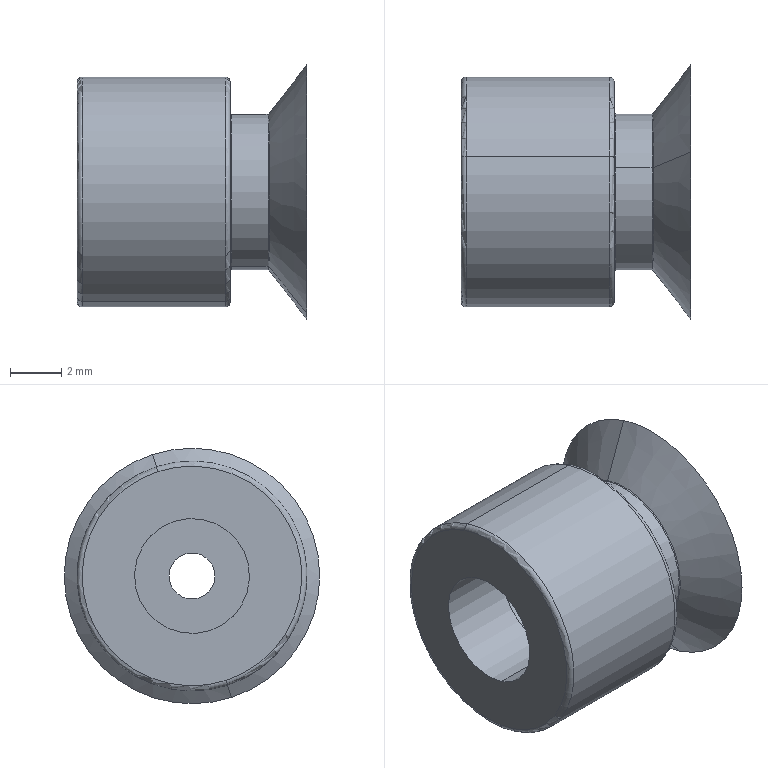Component | SolidWorks | SmallSuctionNozzle-1 | 1 solid | 28 faces | box 9 x 10 x 10 mm | volume 304 mm3 | cylinder 10 | torus 8 | plane 6 | cone 4 | commonest cylinder face diameters 7 x2 1.8 x2 4.5 x2 6.1 x2 9 x2
build123d program:
from build123d import *

# Parameters (mm, degrees)
SKETCH1_R           = 4.5
BOSS_EXTRUDE1_DEPTH = 3
SKETCH2_R           = 3.05
BOSS_EXTRUDE2_DEPTH = 1.5
SKETCH4_R           = 2.25
CUT_EXTRUDE1_DEPTH  = 5.5
SKETCH6_R           = 0.9
CUT_EXTRUDE3_DEPTH  = 11.308
SKETCH7_R           = 3.5
CUT_EXTRUDE6_DEPTH  = 2.5
FILLET1_R           = 0.2
FILLET2_R           = 0.05


with BuildPart() as part:
    # Sketch1 → Boss-Extrude1 (new, symmetric)
    with BuildSketch(Plane.XY):
        Circle(SKETCH1_R)
    extrude(amount=BOSS_EXTRUDE1_DEPTH, both=True)

    # Sketch2 → Boss-Extrude2 (add)
    with BuildSketch(Plane.XY.offset(3)):
        Circle(SKETCH2_R)
    extrude(amount=BOSS_EXTRUDE2_DEPTH)

    # Sketch3 → Revolve1 (revolve)
    with BuildSketch(Plane(origin=(0, 0, 0), x_dir=(1, 0, 0), z_dir=(0, 1, 0)), mode=Mode.PRIVATE) as revolve1_sk:
        Polygon((-4.18, -6), (-2.23, -4.5), (-3.05, -4.5), (-5, -6), align=None)
    revolve(revolve1_sk.sketch.rotate(Axis((0, 0, -3), (0, 0, 1)), 180), axis=Axis((0, 0, -3), (0, 0, 1)))

    # Sketch4 → Cut-Extrude1 (cut)
    with BuildSketch(Plane(origin=(0, 0, -3), x_dir=(-1, 0, 0), z_dir=(0, 0, -1))):
        Circle(SKETCH4_R)
    extrude(amount=-CUT_EXTRUDE1_DEPTH, mode=Mode.SUBTRACT)

    # Sketch6 → Cut-Extrude3 (cut, through all)
    with BuildSketch(Plane.XY.offset(4.5)):
        Circle(SKETCH6_R)
    extrude(amount=-CUT_EXTRUDE3_DEPTH, mode=Mode.SUBTRACT)

    # Sketch7 → Cut-Extrude6 (cut)
    with BuildSketch(Plane(origin=(0, 0, 2.5), x_dir=(-1, 0, 0), z_dir=(0, 0, -1))):
        Circle(SKETCH7_R)
    extrude(amount=CUT_EXTRUDE6_DEPTH, mode=Mode.SUBTRACT)

    # Fillet1
    fillet1_edges = [part.edges().sort_by_distance(p)[0] for p in [
        (-4.5, 0, -3),
        (-4.5, 0, 3),
    ]]
    fillet(fillet1_edges, radius=FILLET1_R)

    # Fillet2
    fillet2_edges = [part.edges().sort_by_distance(p)[0] for p in [
        (-3.05, 0, 3),
        (-3.05, 0, 4.5),
    ]]
    fillet(fillet2_edges, radius=FILLET2_R)


solid = part.part

# Placed as in the assembly
solid = solid.moved(Location((-558.696, -21.651, 373.468), (0, 90, 0)))
STEP:
#1=COLOUR_RGB('',0.7922,0.8196,0.9333);
#2=FILL_AREA_STYLE_COLOUR('',#1);
#3=FILL_AREA_STYLE('',(#2));
#4=SURFACE_STYLE_FILL_AREA(#3);
#5=SURFACE_SIDE_STYLE('',(#4));
#6=SURFACE_STYLE_USAGE(.BOTH.,#5);
#7=PRESENTATION_STYLE_ASSIGNMENT((#6));
#8=CARTESIAN_POINT('',(-21.818,-0.8149,14.818));
#9=VERTEX_POINT('',#8);
#10=CARTESIAN_POINT('',(-21.818,-0.8899,14.589));
#11=VERTEX_POINT('',#10);
#12=CARTESIAN_POINT('',(-21.818,-0.8524,14.703));
#13=DIRECTION('',(1.,-0.,0.));
#14=DIRECTION('',(0.,0.3102,0.9507));
#15=AXIS2_PLACEMENT_3D('',#12,#13,#14);
#16=CIRCLE('',#15,0.1208);
#17=EDGE_CURVE('',#9,#11,#16,.T.);
#18=ORIENTED_EDGE('',*,*,#17,.F.);
#19=CARTESIAN_POINT('',(-21.82,-0.8152,14.818));
#20=VERTEX_POINT('',#19);
#21=CARTESIAN_POINT('',(-21.82,-0.8146,14.819));
#22=DIRECTION('',(0.,0.9507,-0.3102));
#23=DIRECTION('',(0.,0.3102,0.9507));
#24=AXIS2_PLACEMENT_3D('',#21,#22,#23);
#25=CIRCLE('',#24,0.001969);
#26=EDGE_CURVE('',#9,#20,#25,.T.);
#27=ORIENTED_EDGE('',*,*,#26,.T.);
#28=CARTESIAN_POINT('',(-21.82,-0.8897,14.589));
#29=VERTEX_POINT('',#28);
#30=CARTESIAN_POINT('',(-21.82,-0.8524,14.703));
#31=DIRECTION('',(-1.,0.,-0.));
#32=DIRECTION('',(0.,-0.3102,-0.9507));
#33=AXIS2_PLACEMENT_3D('',#30,#31,#32);
#34=CIRCLE('',#33,0.1201);
#35=EDGE_CURVE('',#29,#20,#34,.T.);
#36=ORIENTED_EDGE('',*,*,#35,.F.);
#37=CARTESIAN_POINT('',(-21.82,-0.8903,14.587));
#38=DIRECTION('',(-0.,-0.9507,0.3102));
#39=DIRECTION('',(0.,-0.3102,-0.9507));
#40=AXIS2_PLACEMENT_3D('',#37,#38,#39);
#41=CIRCLE('',#40,0.001969);
#42=EDGE_CURVE('',#11,#29,#41,.T.);
#43=ORIENTED_EDGE('',*,*,#42,.F.);
#44=EDGE_LOOP('',(#18,#27,#36,#43));
#45=FACE_OUTER_BOUND('',#44,.T.);
#46=CARTESIAN_POINT('',(-21.82,-0.8524,14.703));
#47=DIRECTION('',(1.,-0.,0.));
#48=DIRECTION('',(0.,-0.3102,-0.9507));
#49=AXIS2_PLACEMENT_3D('',#46,#47,#48);
#50=TOROIDAL_SURFACE('',#49,0.122,0.001969);
#51=ADVANCED_FACE('',(#45),#50,.F.);
#52=CARTESIAN_POINT('',(-21.876,-0.8152,14.818));
#53=VERTEX_POINT('',#52);
#54=CARTESIAN_POINT('',(-21.876,-0.8897,14.589));
#55=VERTEX_POINT('',#54);
#56=CARTESIAN_POINT('',(-21.876,-0.8524,14.703));
#57=DIRECTION('',(1.,-0.,0.));
#58=DIRECTION('',(0.,-0.3102,-0.9507));
#59=AXIS2_PLACEMENT_3D('',#56,#57,#58);
#60=CIRCLE('',#59,0.1201);
#61=EDGE_CURVE('',#53,#55,#60,.T.);
#62=ORIENTED_EDGE('',*,*,#61,.F.);
#63=CARTESIAN_POINT('',(-21.878,-0.8146,14.819));
#64=VERTEX_POINT('',#63);
#65=CARTESIAN_POINT('',(-21.876,-0.8146,14.819));
#66=DIRECTION('',(0.,0.9507,-0.3102));
#67=DIRECTION('',(0.,0.3102,0.9507));
#68=AXIS2_PLACEMENT_3D('',#65,#66,#67);
#69=CIRCLE('',#68,0.001969);
#70=EDGE_CURVE('',#53,#64,#69,.T.);
#71=ORIENTED_EDGE('',*,*,#70,.T.);
#72=CARTESIAN_POINT('',(-21.878,-0.8903,14.587));
#73=VERTEX_POINT('',#72);
#74=CARTESIAN_POINT('',(-21.878,-0.8524,14.703));
#75=DIRECTION('',(-1.,0.,-0.));
#76=DIRECTION('',(0.,-0.3102,-0.9507));
#77=AXIS2_PLACEMENT_3D('',#74,#75,#76);
#78=CIRCLE('',#77,0.122);
#79=EDGE_CURVE('',#73,#64,#78,.T.);
#80=ORIENTED_EDGE('',*,*,#79,.F.);
#81=CARTESIAN_POINT('',(-21.876,-0.8903,14.587));
#82=DIRECTION('',(-0.,-0.9507,0.3102));
#83=DIRECTION('',(0.,-0.3102,-0.9507));
#84=AXIS2_PLACEMENT_3D('',#81,#82,#83);
#85=CIRCLE('',#84,0.001969);
#86=EDGE_CURVE('',#55,#73,#85,.T.);
#87=ORIENTED_EDGE('',*,*,#86,.F.);
#88=EDGE_LOOP('',(#62,#71,#80,#87));
#89=FACE_OUTER_BOUND('',#88,.T.);
#90=CARTESIAN_POINT('',(-21.876,-0.8524,14.703));
#91=DIRECTION('',(1.,-0.,0.));
#92=DIRECTION('',(0.,-0.3102,-0.9507));
#93=AXIS2_PLACEMENT_3D('',#90,#91,#92);
#94=TOROIDAL_SURFACE('',#93,0.122,0.001969);
#95=ADVANCED_FACE('',(#89),#94,.F.);
#96=CARTESIAN_POINT('',(-21.886,-0.7975,14.872));
#97=VERTEX_POINT('',#96);
#98=CARTESIAN_POINT('',(-21.886,-0.9074,14.535));
#99=VERTEX_POINT('',#98);
#100=CARTESIAN_POINT('',(-21.886,-0.8524,14.703));
#101=DIRECTION('',(-1.,0.,-0.));
#102=DIRECTION('',(0.,-0.3102,-0.9507));
#103=AXIS2_PLACEMENT_3D('',#100,#101,#102);
#104=CIRCLE('',#103,0.1772);
#105=EDGE_CURVE('',#97,#99,#104,.T.);
#106=ORIENTED_EDGE('',*,*,#105,.F.);
#107=CARTESIAN_POINT('',(-21.878,-0.7999,14.864));
#108=VERTEX_POINT('',#107);
#109=CARTESIAN_POINT('',(-21.886,-0.7999,14.864));
#110=DIRECTION('',(0.,0.9507,-0.3102));
#111=DIRECTION('',(0.,0.3102,0.9507));
#112=AXIS2_PLACEMENT_3D('',#109,#110,#111);
#113=CIRCLE('',#112,0.007874);
#114=EDGE_CURVE('',#97,#108,#113,.T.);
#115=ORIENTED_EDGE('',*,*,#114,.T.);
#116=CARTESIAN_POINT('',(-21.878,-0.9049,14.543));
#117=VERTEX_POINT('',#116);
#118=CARTESIAN_POINT('',(-21.878,-0.8524,14.703));
#119=DIRECTION('',(1.,-0.,0.));
#120=DIRECTION('',(0.,-0.3102,-0.9507));
#121=AXIS2_PLACEMENT_3D('',#118,#119,#120);
#122=CIRCLE('',#121,0.1693);
#123=EDGE_CURVE('',#117,#108,#122,.T.);
#124=ORIENTED_EDGE('',*,*,#123,.F.);
#125=CARTESIAN_POINT('',(-21.886,-0.9049,14.543));
#126=DIRECTION('',(-0.,-0.9507,0.3102));
#127=DIRECTION('',(0.,-0.3102,-0.9507));
#128=AXIS2_PLACEMENT_3D('',#125,#126,#127);
#129=CIRCLE('',#128,0.007874);
#130=EDGE_CURVE('',#99,#117,#129,.T.);
#131=ORIENTED_EDGE('',*,*,#130,.F.);
#132=EDGE_LOOP('',(#106,#115,#124,#131));
#133=FACE_OUTER_BOUND('',#132,.T.);
#134=CARTESIAN_POINT('',(-21.886,-0.8524,14.703));
#135=DIRECTION('',(1.,-0.,0.));
#136=DIRECTION('',(0.,-0.3102,-0.9507));
#137=AXIS2_PLACEMENT_3D('',#134,#135,#136);
#138=TOROIDAL_SURFACE('',#137,0.1693,0.007874);
#139=ADVANCED_FACE('',(#133),#138,.T.);
#140=CARTESIAN_POINT('',(-22.114,-0.7999,14.864));
#141=VERTEX_POINT('',#140);
#142=CARTESIAN_POINT('',(-22.114,-0.9049,14.543));
#143=VERTEX_POINT('',#142);
#144=CARTESIAN_POINT('',(-22.114,-0.8524,14.703));
#145=DIRECTION('',(-1.,0.,-0.));
#146=DIRECTION('',(0.,-0.3102,-0.9507));
#147=AXIS2_PLACEMENT_3D('',#144,#145,#146);
#148=CIRCLE('',#147,0.1693);
#149=EDGE_CURVE('',#141,#143,#148,.T.);
#150=ORIENTED_EDGE('',*,*,#149,.F.);
#151=CARTESIAN_POINT('',(-22.106,-0.7975,14.872));
#152=VERTEX_POINT('',#151);
#153=CARTESIAN_POINT('',(-22.106,-0.7999,14.864));
#154=DIRECTION('',(0.,0.9507,-0.3102));
#155=DIRECTION('',(0.,0.3102,0.9507));
#156=AXIS2_PLACEMENT_3D('',#153,#154,#155);
#157=CIRCLE('',#156,0.007874);
#158=EDGE_CURVE('',#141,#152,#157,.T.);
#159=ORIENTED_EDGE('',*,*,#158,.T.);
#160=CARTESIAN_POINT('',(-22.106,-0.9074,14.535));
#161=VERTEX_POINT('',#160);
#162=CARTESIAN_POINT('',(-22.106,-0.8524,14.703));
#163=DIRECTION('',(1.,-0.,0.));
#164=DIRECTION('',(0.,-0.3102,-0.9507));
#165=AXIS2_PLACEMENT_3D('',#162,#163,#164);
#166=CIRCLE('',#165,0.1772);
#167=EDGE_CURVE('',#161,#152,#166,.T.);
#168=ORIENTED_EDGE('',*,*,#167,.F.);
#169=CARTESIAN_POINT('',(-22.106,-0.9049,14.543));
#170=DIRECTION('',(-0.,-0.9507,0.3102));
#171=DIRECTION('',(0.,-0.3102,-0.9507));
#172=AXIS2_PLACEMENT_3D('',#169,#170,#171);
#173=CIRCLE('',#172,0.007874);
#174=EDGE_CURVE('',#143,#161,#173,.T.);
#175=ORIENTED_EDGE('',*,*,#174,.F.);
#176=EDGE_LOOP('',(#150,#159,#168,#175));
#177=FACE_OUTER_BOUND('',#176,.T.);
#178=CARTESIAN_POINT('',(-22.106,-0.8524,14.703));
#179=DIRECTION('',(1.,-0.,0.));
#180=DIRECTION('',(0.,-0.3102,-0.9507));
#181=AXIS2_PLACEMENT_3D('',#178,#179,#180);
#182=TOROIDAL_SURFACE('',#181,0.1693,0.007874);
#183=ADVANCED_FACE('',(#177),#182,.T.);
#184=CARTESIAN_POINT('',(-21.996,-0.8952,14.572));
#185=VERTEX_POINT('',#184);
#186=CARTESIAN_POINT('',(-21.996,-0.8097,14.834));
#187=VERTEX_POINT('',#186);
#188=CARTESIAN_POINT('',(-21.996,-0.8524,14.703));
#189=DIRECTION('',(-1.,0.,-0.));
#190=DIRECTION('',(0.,0.3102,0.9507));
#191=AXIS2_PLACEMENT_3D('',#188,#189,#190);
#192=CIRCLE('',#191,0.1378);
#193=EDGE_CURVE('',#185,#187,#192,.T.);
#194=ORIENTED_EDGE('',*,*,#193,.T.);
#195=CARTESIAN_POINT('',(-21.897,-0.8097,14.834));
#196=VERTEX_POINT('',#195);
#197=CARTESIAN_POINT('',(-21.996,-0.8097,14.834));
#198=DIRECTION('',(1.,-0.,0.));
#199=VECTOR('',#198,39.37);
#200=LINE('',#197,#199);
#201=EDGE_CURVE('',#187,#196,#200,.T.);
#202=ORIENTED_EDGE('',*,*,#201,.T.);
#203=CARTESIAN_POINT('',(-21.897,-0.8952,14.572));
#204=VERTEX_POINT('',#203);
#205=CARTESIAN_POINT('',(-21.897,-0.8524,14.703));
#206=DIRECTION('',(-1.,0.,-0.));
#207=DIRECTION('',(0.,0.3102,0.9507));
#208=AXIS2_PLACEMENT_3D('',#205,#206,#207);
#209=CIRCLE('',#208,0.1378);
#210=EDGE_CURVE('',#204,#196,#209,.T.);
#211=ORIENTED_EDGE('',*,*,#210,.F.);
#212=CARTESIAN_POINT('',(-21.996,-0.8952,14.572));
#213=DIRECTION('',(1.,-0.,0.));
#214=VECTOR('',#213,39.37);
#215=LINE('',#212,#214);
#216=EDGE_CURVE('',#185,#204,#215,.T.);
#217=ORIENTED_EDGE('',*,*,#216,.F.);
#218=EDGE_LOOP('',(#194,#202,#211,#217));
#219=FACE_OUTER_BOUND('',#218,.T.);
#220=CARTESIAN_POINT('',(-21.996,-0.8524,14.703));
#221=DIRECTION('',(1.,-0.,0.));
#222=DIRECTION('',(0.,-0.3102,-0.9507));
#223=AXIS2_PLACEMENT_3D('',#220,#221,#222);
#224=CYLINDRICAL_SURFACE('',#223,0.1378);
#225=ADVANCED_FACE('',(#219),#224,.F.);
#226=CARTESIAN_POINT('',(-21.897,-0.8634,14.67));
#227=VERTEX_POINT('',#226);
#228=CARTESIAN_POINT('',(-21.897,-0.8414,14.737));
#229=VERTEX_POINT('',#228);
#230=CARTESIAN_POINT('',(-21.897,-0.8524,14.703));
#231=DIRECTION('',(-1.,0.,-0.));
#232=DIRECTION('',(0.,0.3102,0.9507));
#233=AXIS2_PLACEMENT_3D('',#230,#231,#232);
#234=CIRCLE('',#233,0.03543);
#235=EDGE_CURVE('',#227,#229,#234,.T.);
#236=ORIENTED_EDGE('',*,*,#235,.T.);
#237=CARTESIAN_POINT('',(-21.819,-0.8414,14.737));
#238=VERTEX_POINT('',#237);
#239=CARTESIAN_POINT('',(-22.114,-0.8414,14.737));
#240=DIRECTION('',(1.,-0.,0.));
#241=VECTOR('',#240,39.37);
#242=LINE('',#239,#241);
#243=EDGE_CURVE('',#229,#238,#242,.T.);
#244=ORIENTED_EDGE('',*,*,#243,.T.);
#245=CARTESIAN_POINT('',(-21.819,-0.8634,14.67));
#246=VERTEX_POINT('',#245);
#247=CARTESIAN_POINT('',(-21.819,-0.8524,14.703));
#248=DIRECTION('',(1.,-0.,0.));
#249=DIRECTION('',(0.,-0.3102,-0.9507));
#250=AXIS2_PLACEMENT_3D('',#247,#248,#249);
#251=CIRCLE('',#250,0.03543);
#252=EDGE_CURVE('',#238,#246,#251,.T.);
#253=ORIENTED_EDGE('',*,*,#252,.T.);
#254=CARTESIAN_POINT('',(-22.114,-0.8634,14.67));
#255=DIRECTION('',(1.,-0.,0.));
#256=VECTOR('',#255,39.37);
#257=LINE('',#254,#256);
#258=EDGE_CURVE('',#227,#246,#257,.T.);
#259=ORIENTED_EDGE('',*,*,#258,.F.);
#260=EDGE_LOOP('',(#236,#244,#253,#259));
#261=FACE_OUTER_BOUND('',#260,.T.);
#262=CARTESIAN_POINT('',(-22.114,-0.8524,14.703));
#263=DIRECTION('',(1.,-0.,0.));
#264=DIRECTION('',(0.,-0.3102,-0.9507));
#265=AXIS2_PLACEMENT_3D('',#262,#263,#264);
#266=CYLINDRICAL_SURFACE('',#265,0.03543);
#267=ADVANCED_FACE('',(#261),#266,.F.);
#268=CARTESIAN_POINT('',(-21.996,-0.8249,14.788));
#269=VERTEX_POINT('',#268);
#270=CARTESIAN_POINT('',(-21.996,-0.8799,14.619));
#271=VERTEX_POINT('',#270);
#272=CARTESIAN_POINT('',(-21.996,-0.8524,14.703));
#273=DIRECTION('',(1.,-0.,0.));
#274=DIRECTION('',(0.,0.3102,0.9507));
#275=AXIS2_PLACEMENT_3D('',#272,#273,#274);
#276=CIRCLE('',#275,0.08858);
#277=EDGE_CURVE('',#269,#271,#276,.T.);
#278=ORIENTED_EDGE('',*,*,#277,.T.);
#279=CARTESIAN_POINT('',(-22.114,-0.8799,14.619));
#280=VERTEX_POINT('',#279);
#281=CARTESIAN_POINT('',(-21.897,-0.8799,14.619));
#282=DIRECTION('',(-1.,0.,-0.));
#283=VECTOR('',#282,39.37);
#284=LINE('',#281,#283);
#285=EDGE_CURVE('',#271,#280,#284,.T.);
#286=ORIENTED_EDGE('',*,*,#285,.T.);
#287=CARTESIAN_POINT('',(-22.114,-0.8249,14.788));
#288=VERTEX_POINT('',#287);
#289=CARTESIAN_POINT('',(-22.114,-0.8524,14.703));
#290=DIRECTION('',(-1.,0.,-0.));
#291=DIRECTION('',(0.,0.3102,0.9507));
#292=AXIS2_PLACEMENT_3D('',#289,#290,#291);
#293=CIRCLE('',#292,0.08858);
#294=EDGE_CURVE('',#280,#288,#293,.T.);
#295=ORIENTED_EDGE('',*,*,#294,.T.);
#296=CARTESIAN_POINT('',(-21.897,-0.8249,14.788));
#297=DIRECTION('',(-1.,0.,-0.));
#298=VECTOR('',#297,39.37);
#299=LINE('',#296,#298);
#300=EDGE_CURVE('',#269,#288,#299,.T.);
#301=ORIENTED_EDGE('',*,*,#300,.F.);
#302=EDGE_LOOP('',(#278,#286,#295,#301));
#303=FACE_OUTER_BOUND('',#302,.T.);
#304=CARTESIAN_POINT('',(-21.897,-0.8524,14.703));
#305=DIRECTION('',(-1.,0.,-0.));
#306=DIRECTION('',(0.,0.3102,0.9507));
#307=AXIS2_PLACEMENT_3D('',#304,#305,#306);
#308=CYLINDRICAL_SURFACE('',#307,0.08858);
#309=ADVANCED_FACE('',(#303),#308,.F.);
#310=CARTESIAN_POINT('',(-21.818,-0.8524,14.703));
#311=DIRECTION('',(1.,-0.,0.));
#312=DIRECTION('',(0.,0.3102,0.9507));
#313=AXIS2_PLACEMENT_3D('',#310,#311,#312);
#314=CIRCLE('',#313,0.1208);
#315=EDGE_CURVE('',#11,#9,#314,.T.);
#316=ORIENTED_EDGE('',*,*,#315,.T.);
#317=CARTESIAN_POINT('',(-21.76,-0.7914,14.891));
#318=VERTEX_POINT('',#317);
#319=CARTESIAN_POINT('',(-21.819,-0.8152,14.818));
#320=DIRECTION('',(0.6097,0.2459,0.7535));
#321=VECTOR('',#320,39.37);
#322=LINE('',#319,#321);
#323=EDGE_CURVE('',#9,#318,#322,.T.);
#324=ORIENTED_EDGE('',*,*,#323,.T.);
#325=CARTESIAN_POINT('',(-21.76,-0.9135,14.516));
#326=VERTEX_POINT('',#325);
#327=CARTESIAN_POINT('',(-21.76,-0.8524,14.703));
#328=DIRECTION('',(-1.,0.,-0.));
#329=DIRECTION('',(0.,0.3102,0.9507));
#330=AXIS2_PLACEMENT_3D('',#327,#328,#329);
#331=CIRCLE('',#330,0.1969);
#332=EDGE_CURVE('',#318,#326,#331,.T.);
#333=ORIENTED_EDGE('',*,*,#332,.T.);
#334=CARTESIAN_POINT('',(-21.819,-0.8897,14.589));
#335=DIRECTION('',(0.6097,-0.2459,-0.7535));
#336=VECTOR('',#335,39.37);
#337=LINE('',#334,#336);
#338=EDGE_CURVE('',#11,#326,#337,.T.);
#339=ORIENTED_EDGE('',*,*,#338,.F.);
#340=EDGE_LOOP('',(#316,#324,#333,#339));
#341=FACE_OUTER_BOUND('',#340,.T.);
#342=CARTESIAN_POINT('',(-21.819,-0.8524,14.703));
#343=DIRECTION('',(1.,-0.,0.));
#344=DIRECTION('',(0.,-0.3102,-0.9507));
#345=AXIS2_PLACEMENT_3D('',#342,#343,#344);
#346=CONICAL_SURFACE('',#345,0.1201,0.9151);
#347=ADVANCED_FACE('',(#341),#346,.T.);
#348=CARTESIAN_POINT('',(-21.819,-0.8796,14.62));
#349=VERTEX_POINT('',#348);
#350=CARTESIAN_POINT('',(-21.819,-0.8252,14.787));
#351=VERTEX_POINT('',#350);
#352=CARTESIAN_POINT('',(-21.819,-0.8524,14.703));
#353=DIRECTION('',(-1.,0.,-0.));
#354=DIRECTION('',(0.,-0.3102,-0.9507));
#355=AXIS2_PLACEMENT_3D('',#352,#353,#354);
#356=CIRCLE('',#355,0.08779);
#357=EDGE_CURVE('',#349,#351,#356,.T.);
#358=ORIENTED_EDGE('',*,*,#357,.T.);
#359=CARTESIAN_POINT('',(-21.76,-0.8014,14.86));
#360=VERTEX_POINT('',#359);
#361=CARTESIAN_POINT('',(-21.76,-0.8014,14.86));
#362=DIRECTION('',(0.6097,0.2459,0.7535));
#363=VECTOR('',#362,39.37);
#364=LINE('',#361,#363);
#365=EDGE_CURVE('',#351,#360,#364,.T.);
#366=ORIENTED_EDGE('',*,*,#365,.T.);
#367=CARTESIAN_POINT('',(-21.76,-0.9035,14.547));
#368=VERTEX_POINT('',#367);
#369=CARTESIAN_POINT('',(-21.76,-0.8524,14.703));
#370=DIRECTION('',(-1.,0.,-0.));
#371=DIRECTION('',(0.,0.3102,0.9507));
#372=AXIS2_PLACEMENT_3D('',#369,#370,#371);
#373=CIRCLE('',#372,0.1646);
#374=EDGE_CURVE('',#368,#360,#373,.T.);
#375=ORIENTED_EDGE('',*,*,#374,.F.);
#376=CARTESIAN_POINT('',(-21.76,-0.9035,14.547));
#377=DIRECTION('',(0.6097,-0.2459,-0.7535));
#378=VECTOR('',#377,39.37);
#379=LINE('',#376,#378);
#380=EDGE_CURVE('',#349,#368,#379,.T.);
#381=ORIENTED_EDGE('',*,*,#380,.F.);
#382=EDGE_LOOP('',(#358,#366,#375,#381));
#383=FACE_OUTER_BOUND('',#382,.T.);
#384=CARTESIAN_POINT('',(-21.76,-0.8524,14.703));
#385=DIRECTION('',(1.,-0.,0.));
#386=DIRECTION('',(0.,-0.3102,-0.9507));
#387=AXIS2_PLACEMENT_3D('',#384,#385,#386);
#388=CONICAL_SURFACE('',#387,0.1646,0.9151);
#389=ADVANCED_FACE('',(#383),#388,.F.);
#390=CARTESIAN_POINT('',(-21.82,-0.8524,14.703));
#391=DIRECTION('',(-1.,0.,-0.));
#392=DIRECTION('',(0.,-0.3102,-0.9507));
#393=AXIS2_PLACEMENT_3D('',#390,#391,#392);
#394=CIRCLE('',#393,0.1201);
#395=EDGE_CURVE('',#20,#29,#394,.T.);
#396=ORIENTED_EDGE('',*,*,#395,.T.);
#397=CARTESIAN_POINT('',(-21.819,-0.8897,14.589));
#398=DIRECTION('',(-1.,0.,-0.));
#399=VECTOR('',#398,39.37);
#400=LINE('',#397,#399);
#401=EDGE_CURVE('',#29,#55,#400,.T.);
#402=ORIENTED_EDGE('',*,*,#401,.T.);
#403=CARTESIAN_POINT('',(-21.876,-0.8524,14.703));
#404=DIRECTION('',(1.,-0.,0.));
#405=DIRECTION('',(0.,-0.3102,-0.9507));
#406=AXIS2_PLACEMENT_3D('',#403,#404,#405);
#407=CIRCLE('',#406,0.1201);
#408=EDGE_CURVE('',#55,#53,#407,.T.);
#409=ORIENTED_EDGE('',*,*,#408,.T.);
#410=CARTESIAN_POINT('',(-21.819,-0.8152,14.818));
#411=DIRECTION('',(-1.,0.,-0.));
#412=VECTOR('',#411,39.37);
#413=LINE('',#410,#412);
#414=EDGE_CURVE('',#20,#53,#413,.T.);
#415=ORIENTED_EDGE('',*,*,#414,.F.);
#416=EDGE_LOOP('',(#396,#402,#409,#415));
#417=FACE_OUTER_BOUND('',#416,.T.);
#418=CARTESIAN_POINT('',(-21.819,-0.8524,14.703));
#419=DIRECTION('',(-1.,0.,-0.));
#420=DIRECTION('',(0.,0.3102,0.9507));
#421=AXIS2_PLACEMENT_3D('',#418,#419,#420);
#422=CYLINDRICAL_SURFACE('',#421,0.1201);
#423=ADVANCED_FACE('',(#417),#422,.T.);
#424=ORIENTED_EDGE('',*,*,#105,.T.);
#425=CARTESIAN_POINT('',(-21.878,-0.9074,14.535));
#426=DIRECTION('',(-1.,0.,-0.));
#427=VECTOR('',#426,39.37);
#428=LINE('',#425,#427);
#429=EDGE_CURVE('',#99,#161,#428,.T.);
#430=ORIENTED_EDGE('',*,*,#429,.T.);
#431=ORIENTED_EDGE('',*,*,#167,.T.);
#432=CARTESIAN_POINT('',(-21.878,-0.7975,14.872));
#433=DIRECTION('',(-1.,0.,-0.));
#434=VECTOR('',#433,39.37);
#435=LINE('',#432,#434);
#436=EDGE_CURVE('',#97,#152,#435,.T.);
#437=ORIENTED_EDGE('',*,*,#436,.F.);
#438=EDGE_LOOP('',(#424,#430,#431,#437));
#439=FACE_OUTER_BOUND('',#438,.T.);
#440=CARTESIAN_POINT('',(-21.878,-0.8524,14.703));
#441=DIRECTION('',(-1.,0.,-0.));
#442=DIRECTION('',(0.,0.3102,0.9507));
#443=AXIS2_PLACEMENT_3D('',#440,#441,#442);
#444=CYLINDRICAL_SURFACE('',#443,0.1772);
#445=ADVANCED_FACE('',(#439),#444,.T.);
#446=ORIENTED_EDGE('',*,*,#79,.T.);
#447=CARTESIAN_POINT('',(-21.878,-0.8524,14.703));
#448=DIRECTION('',(-1.,0.,-0.));
#449=DIRECTION('',(0.,-0.3102,-0.9507));
#450=AXIS2_PLACEMENT_3D('',#447,#448,#449);
#451=CIRCLE('',#450,0.122);
#452=EDGE_CURVE('',#64,#73,#451,.T.);
#453=ORIENTED_EDGE('',*,*,#452,.T.);
#454=EDGE_LOOP('',(#446,#453));
#455=FACE_BOUND('',#454,.T.);
#456=ORIENTED_EDGE('',*,*,#123,.T.);
#457=CARTESIAN_POINT('',(-21.878,-0.8524,14.703));
#458=DIRECTION('',(1.,-0.,0.));
#459=DIRECTION('',(0.,-0.3102,-0.9507));
#460=AXIS2_PLACEMENT_3D('',#457,#458,#459);
#461=CIRCLE('',#460,0.1693);
#462=EDGE_CURVE('',#108,#117,#461,.T.);
#463=ORIENTED_EDGE('',*,*,#462,.T.);
#464=EDGE_LOOP('',(#456,#463));
#465=FACE_OUTER_BOUND('',#464,.T.);
#466=CARTESIAN_POINT('',(-21.878,-0.8524,14.703));
#467=DIRECTION('',(1.,0.,0.));
#468=DIRECTION('',(0.,-0.3102,-0.9507));
#469=AXIS2_PLACEMENT_3D('',#466,#467,#468);
#470=PLANE('',#469);
#471=ADVANCED_FACE('',(#455,#465),#470,.T.);
#472=ORIENTED_EDGE('',*,*,#429,.F.);
#473=CARTESIAN_POINT('',(-21.886,-0.8524,14.703));
#474=DIRECTION('',(-1.,0.,-0.));
#475=DIRECTION('',(0.,-0.3102,-0.9507));
#476=AXIS2_PLACEMENT_3D('',#473,#474,#475);
#477=CIRCLE('',#476,0.1772);
#478=EDGE_CURVE('',#99,#97,#477,.T.);
#479=ORIENTED_EDGE('',*,*,#478,.T.);
#480=ORIENTED_EDGE('',*,*,#436,.T.);
#481=CARTESIAN_POINT('',(-22.106,-0.8524,14.703));
#482=DIRECTION('',(1.,-0.,0.));
#483=DIRECTION('',(0.,-0.3102,-0.9507));
#484=AXIS2_PLACEMENT_3D('',#481,#482,#483);
#485=CIRCLE('',#484,0.1772);
#486=EDGE_CURVE('',#152,#161,#485,.T.);
#487=ORIENTED_EDGE('',*,*,#486,.T.);
#488=EDGE_LOOP('',(#472,#479,#480,#487));
#489=FACE_OUTER_BOUND('',#488,.T.);
#490=CARTESIAN_POINT('',(-21.878,-0.8524,14.703));
#491=DIRECTION('',(-1.,0.,-0.));
#492=DIRECTION('',(0.,0.3102,0.9507));
#493=AXIS2_PLACEMENT_3D('',#490,#491,#492);
#494=CYLINDRICAL_SURFACE('',#493,0.1772);
#495=ADVANCED_FACE('',(#489),#494,.T.);
#496=CARTESIAN_POINT('',(-22.114,-0.8524,14.703));
#497=DIRECTION('',(-1.,0.,-0.));
#498=DIRECTION('',(0.,-0.3102,-0.9507));
#499=AXIS2_PLACEMENT_3D('',#496,#497,#498);
#500=CIRCLE('',#499,0.1693);
#501=EDGE_CURVE('',#143,#141,#500,.T.);
#502=ORIENTED_EDGE('',*,*,#501,.T.);
#503=ORIENTED_EDGE('',*,*,#149,.T.);
#504=EDGE_LOOP('',(#502,#503));
#505=FACE_OUTER_BOUND('',#504,.T.);
#506=CARTESIAN_POINT('',(-22.114,-0.8524,14.703));
#507=DIRECTION('',(-1.,0.,-0.));
#508=DIRECTION('',(0.,0.3102,0.9507));
#509=AXIS2_PLACEMENT_3D('',#506,#507,#508);
#510=CIRCLE('',#509,0.08858);
#511=EDGE_CURVE('',#288,#280,#510,.T.);
#512=ORIENTED_EDGE('',*,*,#511,.F.);
#513=ORIENTED_EDGE('',*,*,#294,.F.);
#514=EDGE_LOOP('',(#512,#513));
#515=FACE_BOUND('',#514,.T.);
#516=CARTESIAN_POINT('',(-22.114,-0.8524,14.703));
#517=DIRECTION('',(1.,0.,0.));
#518=DIRECTION('',(0.,-0.3102,-0.9507));
#519=AXIS2_PLACEMENT_3D('',#516,#517,#518);
#520=PLANE('',#519);
#521=ADVANCED_FACE('',(#505,#515),#520,.F.);
#522=ORIENTED_EDGE('',*,*,#401,.F.);
#523=ORIENTED_EDGE('',*,*,#35,.T.);
#524=ORIENTED_EDGE('',*,*,#414,.T.);
#525=ORIENTED_EDGE('',*,*,#61,.T.);
#526=EDGE_LOOP('',(#522,#523,#524,#525));
#527=FACE_OUTER_BOUND('',#526,.T.);
#528=CARTESIAN_POINT('',(-21.819,-0.8524,14.703));
#529=DIRECTION('',(-1.,0.,-0.));
#530=DIRECTION('',(0.,0.3102,0.9507));
#531=AXIS2_PLACEMENT_3D('',#528,#529,#530);
#532=CYLINDRICAL_SURFACE('',#531,0.1201);
#533=ADVANCED_FACE('',(#527),#532,.T.);
#534=ORIENTED_EDGE('',*,*,#374,.T.);
#535=CARTESIAN_POINT('',(-21.76,-0.8524,14.703));
#536=DIRECTION('',(-1.,0.,-0.));
#537=DIRECTION('',(0.,0.3102,0.9507));
#538=AXIS2_PLACEMENT_3D('',#535,#536,#537);
#539=CIRCLE('',#538,0.1646);
#540=EDGE_CURVE('',#360,#368,#539,.T.);
#541=ORIENTED_EDGE('',*,*,#540,.T.);
#542=EDGE_LOOP('',(#534,#541));
#543=FACE_BOUND('',#542,.T.);
#544=CARTESIAN_POINT('',(-21.76,-0.8524,14.703));
#545=DIRECTION('',(-1.,0.,-0.));
#546=DIRECTION('',(0.,0.3102,0.9507));
#547=AXIS2_PLACEMENT_3D('',#544,#545,#546);
#548=CIRCLE('',#547,0.1969);
#549=EDGE_CURVE('',#326,#318,#548,.T.);
#550=ORIENTED_EDGE('',*,*,#549,.F.);
#551=ORIENTED_EDGE('',*,*,#332,.F.);
#552=EDGE_LOOP('',(#550,#551));
#553=FACE_OUTER_BOUND('',#552,.T.);
#554=CARTESIAN_POINT('',(-21.76,-0.7914,14.891));
#555=DIRECTION('',(1.,0.,0.));
#556=DIRECTION('',(0.,-0.3102,-0.9507));
#557=AXIS2_PLACEMENT_3D('',#554,#555,#556);
#558=PLANE('',#557);
#559=ADVANCED_FACE('',(#543,#553),#558,.T.);
#560=ORIENTED_EDGE('',*,*,#365,.F.);
#561=CARTESIAN_POINT('',(-21.819,-0.8524,14.703));
#562=DIRECTION('',(-1.,0.,-0.));
#563=DIRECTION('',(0.,-0.3102,-0.9507));
#564=AXIS2_PLACEMENT_3D('',#561,#562,#563);
#565=CIRCLE('',#564,0.08779);
#566=EDGE_CURVE('',#351,#349,#565,.T.);
#567=ORIENTED_EDGE('',*,*,#566,.T.);
#568=ORIENTED_EDGE('',*,*,#380,.T.);
#569=ORIENTED_EDGE('',*,*,#540,.F.);
#570=EDGE_LOOP('',(#560,#567,#568,#569));
#571=FACE_OUTER_BOUND('',#570,.T.);
#572=CARTESIAN_POINT('',(-21.76,-0.8524,14.703));
#573=DIRECTION('',(1.,-0.,0.));
#574=DIRECTION('',(0.,-0.3102,-0.9507));
#575=AXIS2_PLACEMENT_3D('',#572,#573,#574);
#576=CONICAL_SURFACE('',#575,0.1646,0.9151);
#577=ADVANCED_FACE('',(#571),#576,.F.);
#578=ORIENTED_EDGE('',*,*,#323,.F.);
#579=ORIENTED_EDGE('',*,*,#17,.T.);
#580=ORIENTED_EDGE('',*,*,#338,.T.);
#581=ORIENTED_EDGE('',*,*,#549,.T.);
#582=EDGE_LOOP('',(#578,#579,#580,#581));
#583=FACE_OUTER_BOUND('',#582,.T.);
#584=CARTESIAN_POINT('',(-21.819,-0.8524,14.703));
#585=DIRECTION('',(1.,-0.,0.));
#586=DIRECTION('',(0.,-0.3102,-0.9507));
#587=AXIS2_PLACEMENT_3D('',#584,#585,#586);
#588=CONICAL_SURFACE('',#587,0.1201,0.9151);
#589=ADVANCED_FACE('',(#583),#588,.T.);
#590=CARTESIAN_POINT('',(-21.819,-0.8524,14.703));
#591=DIRECTION('',(1.,-0.,0.));
#592=DIRECTION('',(0.,-0.3102,-0.9507));
#593=AXIS2_PLACEMENT_3D('',#590,#591,#592);
#594=CIRCLE('',#593,0.03543);
#595=EDGE_CURVE('',#246,#238,#594,.T.);
#596=ORIENTED_EDGE('',*,*,#595,.F.);
#597=ORIENTED_EDGE('',*,*,#252,.F.);
#598=EDGE_LOOP('',(#596,#597));
#599=FACE_BOUND('',#598,.T.);
#600=ORIENTED_EDGE('',*,*,#357,.F.);
#601=ORIENTED_EDGE('',*,*,#566,.F.);
#602=EDGE_LOOP('',(#600,#601));
#603=FACE_OUTER_BOUND('',#602,.T.);
#604=CARTESIAN_POINT('',(-21.819,-0.8524,14.703));
#605=DIRECTION('',(1.,0.,0.));
#606=DIRECTION('',(0.,-0.3102,-0.9507));
#607=AXIS2_PLACEMENT_3D('',#604,#605,#606);
#608=PLANE('',#607);
#609=ADVANCED_FACE('',(#599,#603),#608,.T.);
#610=ORIENTED_EDGE('',*,*,#285,.F.);
#611=CARTESIAN_POINT('',(-21.996,-0.8524,14.703));
#612=DIRECTION('',(1.,-0.,0.));
#613=DIRECTION('',(0.,0.3102,0.9507));
#614=AXIS2_PLACEMENT_3D('',#611,#612,#613);
#615=CIRCLE('',#614,0.08858);
#616=EDGE_CURVE('',#271,#269,#615,.T.);
#617=ORIENTED_EDGE('',*,*,#616,.T.);
#618=ORIENTED_EDGE('',*,*,#300,.T.);
#619=ORIENTED_EDGE('',*,*,#511,.T.);
#620=EDGE_LOOP('',(#610,#617,#618,#619));
#621=FACE_OUTER_BOUND('',#620,.T.);
#622=CARTESIAN_POINT('',(-21.897,-0.8524,14.703));
#623=DIRECTION('',(-1.,0.,-0.));
#624=DIRECTION('',(0.,0.3102,0.9507));
#625=AXIS2_PLACEMENT_3D('',#622,#623,#624);
#626=CYLINDRICAL_SURFACE('',#625,0.08858);
#627=ADVANCED_FACE('',(#621),#626,.F.);
#628=ORIENTED_EDGE('',*,*,#235,.F.);
#629=CARTESIAN_POINT('',(-21.897,-0.8524,14.703));
#630=DIRECTION('',(-1.,0.,-0.));
#631=DIRECTION('',(0.,0.3102,0.9507));
#632=AXIS2_PLACEMENT_3D('',#629,#630,#631);
#633=CIRCLE('',#632,0.03543);
#634=EDGE_CURVE('',#229,#227,#633,.T.);
#635=ORIENTED_EDGE('',*,*,#634,.F.);
#636=EDGE_LOOP('',(#628,#635));
#637=FACE_BOUND('',#636,.T.);
#638=ORIENTED_EDGE('',*,*,#210,.T.);
#639=CARTESIAN_POINT('',(-21.897,-0.8524,14.703));
#640=DIRECTION('',(-1.,0.,-0.));
#641=DIRECTION('',(0.,0.3102,0.9507));
#642=AXIS2_PLACEMENT_3D('',#639,#640,#641);
#643=CIRCLE('',#642,0.1378);
#644=EDGE_CURVE('',#196,#204,#643,.T.);
#645=ORIENTED_EDGE('',*,*,#644,.T.);
#646=EDGE_LOOP('',(#638,#645));
#647=FACE_OUTER_BOUND('',#646,.T.);
#648=CARTESIAN_POINT('',(-21.897,-0.8524,14.703));
#649=DIRECTION('',(-1.,-0.,-0.));
#650=DIRECTION('',(-0.,0.3102,0.9507));
#651=AXIS2_PLACEMENT_3D('',#648,#649,#650);
#652=PLANE('',#651);
#653=ADVANCED_FACE('',(#637,#647),#652,.T.);
#654=ORIENTED_EDGE('',*,*,#243,.F.);
#655=ORIENTED_EDGE('',*,*,#634,.T.);
#656=ORIENTED_EDGE('',*,*,#258,.T.);
#657=ORIENTED_EDGE('',*,*,#595,.T.);
#658=EDGE_LOOP('',(#654,#655,#656,#657));
#659=FACE_OUTER_BOUND('',#658,.T.);
#660=CARTESIAN_POINT('',(-22.114,-0.8524,14.703));
#661=DIRECTION('',(1.,-0.,0.));
#662=DIRECTION('',(0.,-0.3102,-0.9507));
#663=AXIS2_PLACEMENT_3D('',#660,#661,#662);
#664=CYLINDRICAL_SURFACE('',#663,0.03543);
#665=ADVANCED_FACE('',(#659),#664,.F.);
#666=ORIENTED_EDGE('',*,*,#193,.F.);
#667=CARTESIAN_POINT('',(-21.996,-0.8524,14.703));
#668=DIRECTION('',(-1.,0.,-0.));
#669=DIRECTION('',(0.,0.3102,0.9507));
#670=AXIS2_PLACEMENT_3D('',#667,#668,#669);
#671=CIRCLE('',#670,0.1378);
#672=EDGE_CURVE('',#187,#185,#671,.T.);
#673=ORIENTED_EDGE('',*,*,#672,.F.);
#674=EDGE_LOOP('',(#666,#673));
#675=FACE_OUTER_BOUND('',#674,.T.);
#676=ORIENTED_EDGE('',*,*,#277,.F.);
#677=ORIENTED_EDGE('',*,*,#616,.F.);
#678=EDGE_LOOP('',(#676,#677));
#679=FACE_BOUND('',#678,.T.);
#680=CARTESIAN_POINT('',(-21.996,-0.8524,14.703));
#681=DIRECTION('',(-1.,-0.,-0.));
#682=DIRECTION('',(-0.,0.3102,0.9507));
#683=AXIS2_PLACEMENT_3D('',#680,#681,#682);
#684=PLANE('',#683);
#685=ADVANCED_FACE('',(#675,#679),#684,.F.);
#686=ORIENTED_EDGE('',*,*,#201,.F.);
#687=ORIENTED_EDGE('',*,*,#672,.T.);
#688=ORIENTED_EDGE('',*,*,#216,.T.);
#689=ORIENTED_EDGE('',*,*,#644,.F.);
#690=EDGE_LOOP('',(#686,#687,#688,#689));
#691=FACE_OUTER_BOUND('',#690,.T.);
#692=CARTESIAN_POINT('',(-21.996,-0.8524,14.703));
#693=DIRECTION('',(1.,-0.,0.));
#694=DIRECTION('',(0.,-0.3102,-0.9507));
#695=AXIS2_PLACEMENT_3D('',#692,#693,#694);
#696=CYLINDRICAL_SURFACE('',#695,0.1378);
#697=ADVANCED_FACE('',(#691),#696,.F.);
#698=ORIENTED_EDGE('',*,*,#158,.F.);
#699=ORIENTED_EDGE('',*,*,#501,.F.);
#700=ORIENTED_EDGE('',*,*,#174,.T.);
#701=ORIENTED_EDGE('',*,*,#486,.F.);
#702=EDGE_LOOP('',(#698,#699,#700,#701));
#703=FACE_OUTER_BOUND('',#702,.T.);
#704=CARTESIAN_POINT('',(-22.106,-0.8524,14.703));
#705=DIRECTION('',(1.,-0.,0.));
#706=DIRECTION('',(0.,-0.3102,-0.9507));
#707=AXIS2_PLACEMENT_3D('',#704,#705,#706);
#708=TOROIDAL_SURFACE('',#707,0.1693,0.007874);
#709=ADVANCED_FACE('',(#703),#708,.T.);
#710=ORIENTED_EDGE('',*,*,#114,.F.);
#711=ORIENTED_EDGE('',*,*,#478,.F.);
#712=ORIENTED_EDGE('',*,*,#130,.T.);
#713=ORIENTED_EDGE('',*,*,#462,.F.);
#714=EDGE_LOOP('',(#710,#711,#712,#713));
#715=FACE_OUTER_BOUND('',#714,.T.);
#716=CARTESIAN_POINT('',(-21.886,-0.8524,14.703));
#717=DIRECTION('',(1.,-0.,0.));
#718=DIRECTION('',(0.,-0.3102,-0.9507));
#719=AXIS2_PLACEMENT_3D('',#716,#717,#718);
#720=TOROIDAL_SURFACE('',#719,0.1693,0.007874);
#721=ADVANCED_FACE('',(#715),#720,.T.);
#722=ORIENTED_EDGE('',*,*,#70,.F.);
#723=ORIENTED_EDGE('',*,*,#408,.F.);
#724=ORIENTED_EDGE('',*,*,#86,.T.);
#725=ORIENTED_EDGE('',*,*,#452,.F.);
#726=EDGE_LOOP('',(#722,#723,#724,#725));
#727=FACE_OUTER_BOUND('',#726,.T.);
#728=CARTESIAN_POINT('',(-21.876,-0.8524,14.703));
#729=DIRECTION('',(1.,-0.,0.));
#730=DIRECTION('',(0.,-0.3102,-0.9507));
#731=AXIS2_PLACEMENT_3D('',#728,#729,#730);
#732=TOROIDAL_SURFACE('',#731,0.122,0.001969);
#733=ADVANCED_FACE('',(#727),#732,.F.);
#734=ORIENTED_EDGE('',*,*,#26,.F.);
#735=ORIENTED_EDGE('',*,*,#315,.F.);
#736=ORIENTED_EDGE('',*,*,#42,.T.);
#737=ORIENTED_EDGE('',*,*,#395,.F.);
#738=EDGE_LOOP('',(#734,#735,#736,#737));
#739=FACE_OUTER_BOUND('',#738,.T.);
#740=CARTESIAN_POINT('',(-21.82,-0.8524,14.703));
#741=DIRECTION('',(1.,-0.,0.));
#742=DIRECTION('',(0.,-0.3102,-0.9507));
#743=AXIS2_PLACEMENT_3D('',#740,#741,#742);
#744=TOROIDAL_SURFACE('',#743,0.122,0.001969);
#745=ADVANCED_FACE('',(#739),#744,.F.);
#746=CLOSED_SHELL('',(#51,#95,#139,#183,#225,#267,#309,#347,#389,#423,#445,#471,#495,#521,#533,#559,#577,#589,#609,#627,#653,#665,#685,#697,#709,#721,#733,#745));
#747=MANIFOLD_SOLID_BREP('',#746);
#748=STYLED_ITEM('',(#7),#747);
#749=(LENGTH_UNIT()NAMED_UNIT(*)SI_UNIT($,.METRE.));
#750=LENGTH_MEASURE_WITH_UNIT(LENGTH_MEASURE(0.0254),#749);
#751=DIMENSIONAL_EXPONENTS(1.,0.,0.,0.,0.,0.,0.);
#752=(CONVERSION_BASED_UNIT('',#750)LENGTH_UNIT()NAMED_UNIT(#751));
#753=UNCERTAINTY_MEASURE_WITH_UNIT(LENGTH_MEASURE(0.00001),#752,'','');
#754=(NAMED_UNIT(*)PLANE_ANGLE_UNIT()SI_UNIT($,.RADIAN.));
#755=(NAMED_UNIT(*)SI_UNIT($,.STERADIAN.)SOLID_ANGLE_UNIT());
#756=(GEOMETRIC_REPRESENTATION_CONTEXT(3)GLOBAL_UNCERTAINTY_ASSIGNED_CONTEXT((#753))GLOBAL_UNIT_ASSIGNED_CONTEXT((#752,#754,#755))REPRESENTATION_CONTEXT('',''));
#757=MECHANICAL_DESIGN_GEOMETRIC_PRESENTATION_REPRESENTATION('',(#748),#756);
#758=PRESENTATION_LAYER_ASSIGNMENT('','',(#748));
#759=CARTESIAN_POINT('',(0.,0.,0.));
#760=DIRECTION('',(0.,0.,1.));
#761=DIRECTION('',(1.,0.,0.));
#762=AXIS2_PLACEMENT_3D('',#759,#760,#761);
#763=(LENGTH_UNIT()NAMED_UNIT(*)SI_UNIT($,.METRE.));
#764=LENGTH_MEASURE_WITH_UNIT(LENGTH_MEASURE(0.0254),#763);
#765=DIMENSIONAL_EXPONENTS(1.,0.,0.,0.,0.,0.,0.);
#766=(CONVERSION_BASED_UNIT('',#764)LENGTH_UNIT()NAMED_UNIT(#765));
#767=UNCERTAINTY_MEASURE_WITH_UNIT(LENGTH_MEASURE(0.00001),#766,'','');
#768=(NAMED_UNIT(*)PLANE_ANGLE_UNIT()SI_UNIT($,.RADIAN.));
#769=(NAMED_UNIT(*)SI_UNIT($,.STERADIAN.)SOLID_ANGLE_UNIT());
#770=(GEOMETRIC_REPRESENTATION_CONTEXT(3)GLOBAL_UNCERTAINTY_ASSIGNED_CONTEXT((#767))GLOBAL_UNIT_ASSIGNED_CONTEXT((#766,#768,#769))REPRESENTATION_CONTEXT('',''));
#771=ADVANCED_BREP_SHAPE_REPRESENTATION('',(#747,#762),#770);